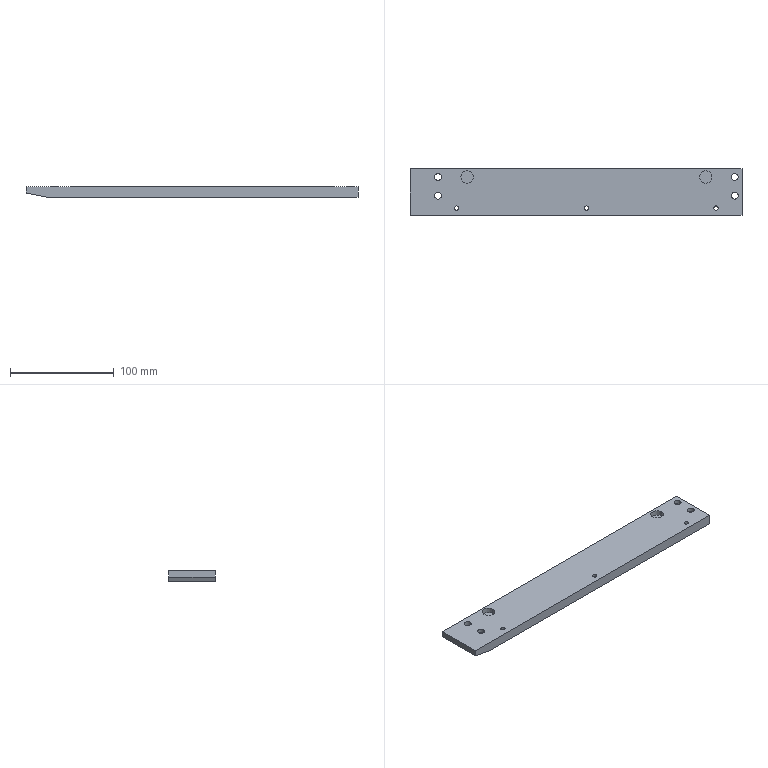Component | SolidWorks | STB-08-005-1 | 1 solid | 39 faces | box 320 x 45 x 10 mm | volume 137825 mm3 | cylinder 26 | plane 13 | commonest cylinder face diameters 11 x8 6.6 x8 4.2 x6 12 x4
build123d program:
from build123d import *

# Parameters (mm, degrees)
SKETCH1_W                                       = 320
SKETCH1_H                                       = 45
BOSS_EXTRUDE1_DEPTH                             = 5
CUT_EXTRUDE1_REACH                              = 168.283
M6_HEX_SOCKET_HEAD_CAP_SCREW_CBORE1_D           = 6.6
M6_HEX_SOCKET_HEAD_CAP_SCREW_CBORE1_CBORE_D     = 11
M6_HEX_SOCKET_HEAD_CAP_SCREW_CBORE1_CBORE_DEPTH = 6
M5_TAPPED_HOLE1_D                               = 4.2
M5_TAPPED_HOLE1_DEPTH                           = 14
M5_TAPPED_HOLE1_TIP                             = 1.262
SKETCH7_R                                       = 6
CUT_EXTRUDE2_DEPTH                              = 5


with BuildPart() as part:
    # Sketch1 → Boss-Extrude1 (new, symmetric)
    with BuildSketch(Plane.XY):
        Rectangle(SKETCH1_W, SKETCH1_H)
    extrude(amount=BOSS_EXTRUDE1_DEPTH, both=True)

    # Sketch2 → Cut-Extrude1 (cut, up to next)
    with BuildSketch(Plane(origin=(0, 22.5, 0), x_dir=(1, 0, 0), z_dir=(0, 1, 0)), mode=Mode.PRIVATE) as cut_extrude1_sk1:
        Polygon((160, -1), (140, -5), (160, -5), align=None)
    cut_extrude1_tool1 = extrude(cut_extrude1_sk1.sketch, amount=-CUT_EXTRUDE1_REACH, mode=Mode.PRIVATE) & part.part
    add(cut_extrude1_tool1.solids().sort_by_distance((153.333, 22.5, 3.667))[0], mode=Mode.SUBTRACT)

    # M6 Hex Socket Head Cap Screw CBORE1 (through all)
    with Locations(Plane.XY.offset(5)):
        with Locations((-153, 14.5), (-153, -3.5), (133, 14.5), (133, -3.5)):
            CounterBoreHole(M6_HEX_SOCKET_HEAD_CAP_SCREW_CBORE1_D / 2, M6_HEX_SOCKET_HEAD_CAP_SCREW_CBORE1_CBORE_D / 2, M6_HEX_SOCKET_HEAD_CAP_SCREW_CBORE1_CBORE_DEPTH)

    # M5 Tapped Hole1
    with Locations(Plane.XY.offset(5)):
        with Locations((-135, -15.5), (-10, -15.5), (115, -15.5)):
            Hole(M5_TAPPED_HOLE1_D / 2, depth=M5_TAPPED_HOLE1_DEPTH)
            with Locations((0, 0, -(M5_TAPPED_HOLE1_DEPTH + M5_TAPPED_HOLE1_TIP / 2))):  # 118° drill point
                Cone(0, M5_TAPPED_HOLE1_D / 2, M5_TAPPED_HOLE1_TIP, mode=Mode.SUBTRACT)

    # Sketch7 → Cut-Extrude2 (cut)
    with BuildSketch(Plane(origin=(0, 0, -5), x_dir=(-1, 0, 0), z_dir=(0, 0, -1))):
        with Locations((125, 14.5)):
            Circle(SKETCH7_R)
        with Locations((-105, 14.5)):
            Circle(SKETCH7_R)
    extrude(amount=-CUT_EXTRUDE2_DEPTH, mode=Mode.SUBTRACT)


solid = part.part

# Placed as in the assembly
solid = solid.moved(Location((-114.904, 76.499, -35), (-180, 0, 180)))